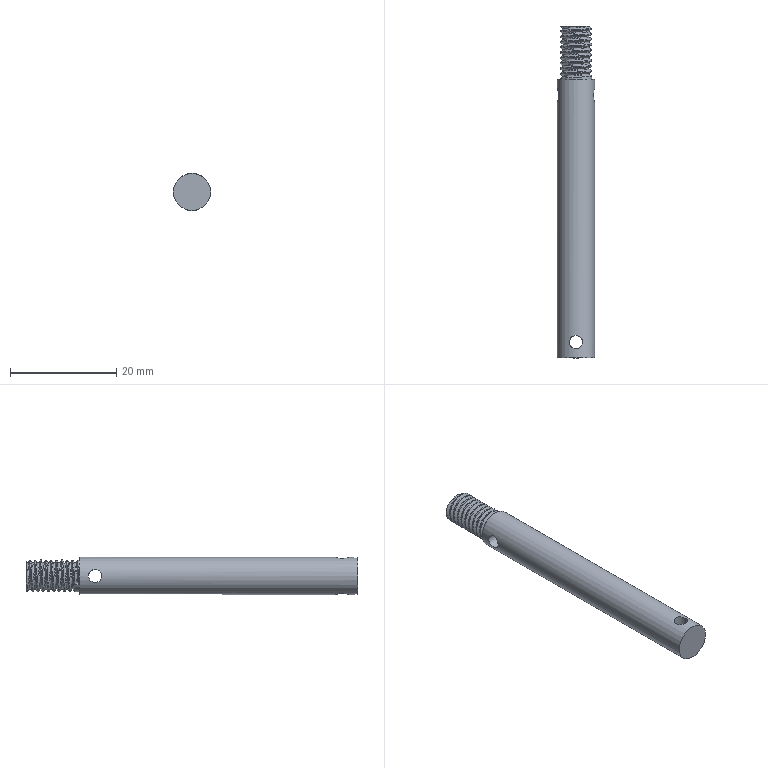Component | NX | XIAO | 1 solid | 12 faces | volume 2184 mm3 | cylinder 5 | plane 4 | spline 3 | commonest cylinder face diameters 2.5 x2 7 x1 6 x1 5 x1